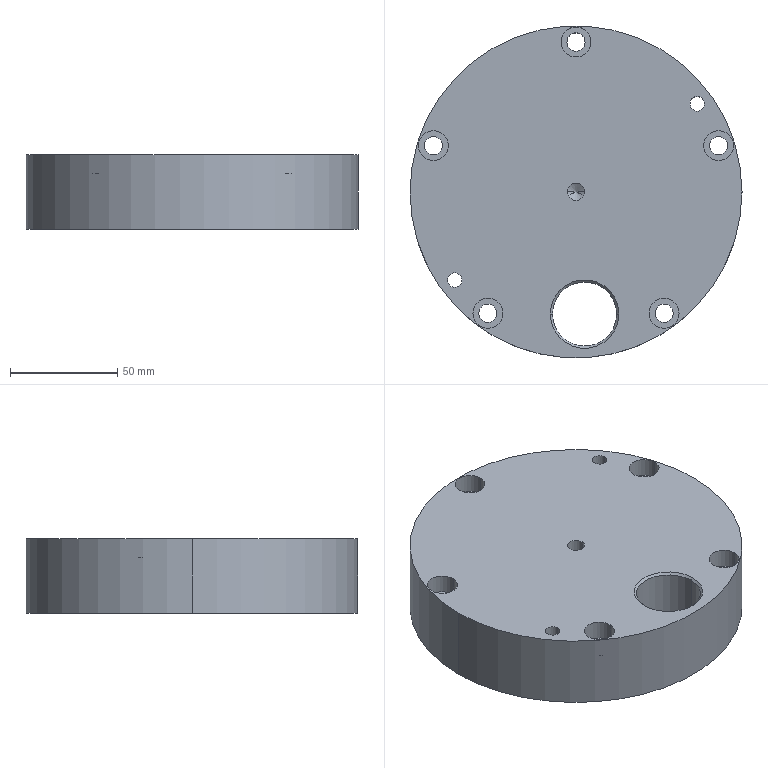Component | SolidWorks | 14FrontFlange-1 | 1 solid | 77 faces | volume 341817 mm3 | cylinder 63 | plane 8 | cone 6 | commonest cylinder face diameters 10 x17 14 x10 8.5 x10 20 x9 130 x6 6.8 x4 8 x2 30 x2